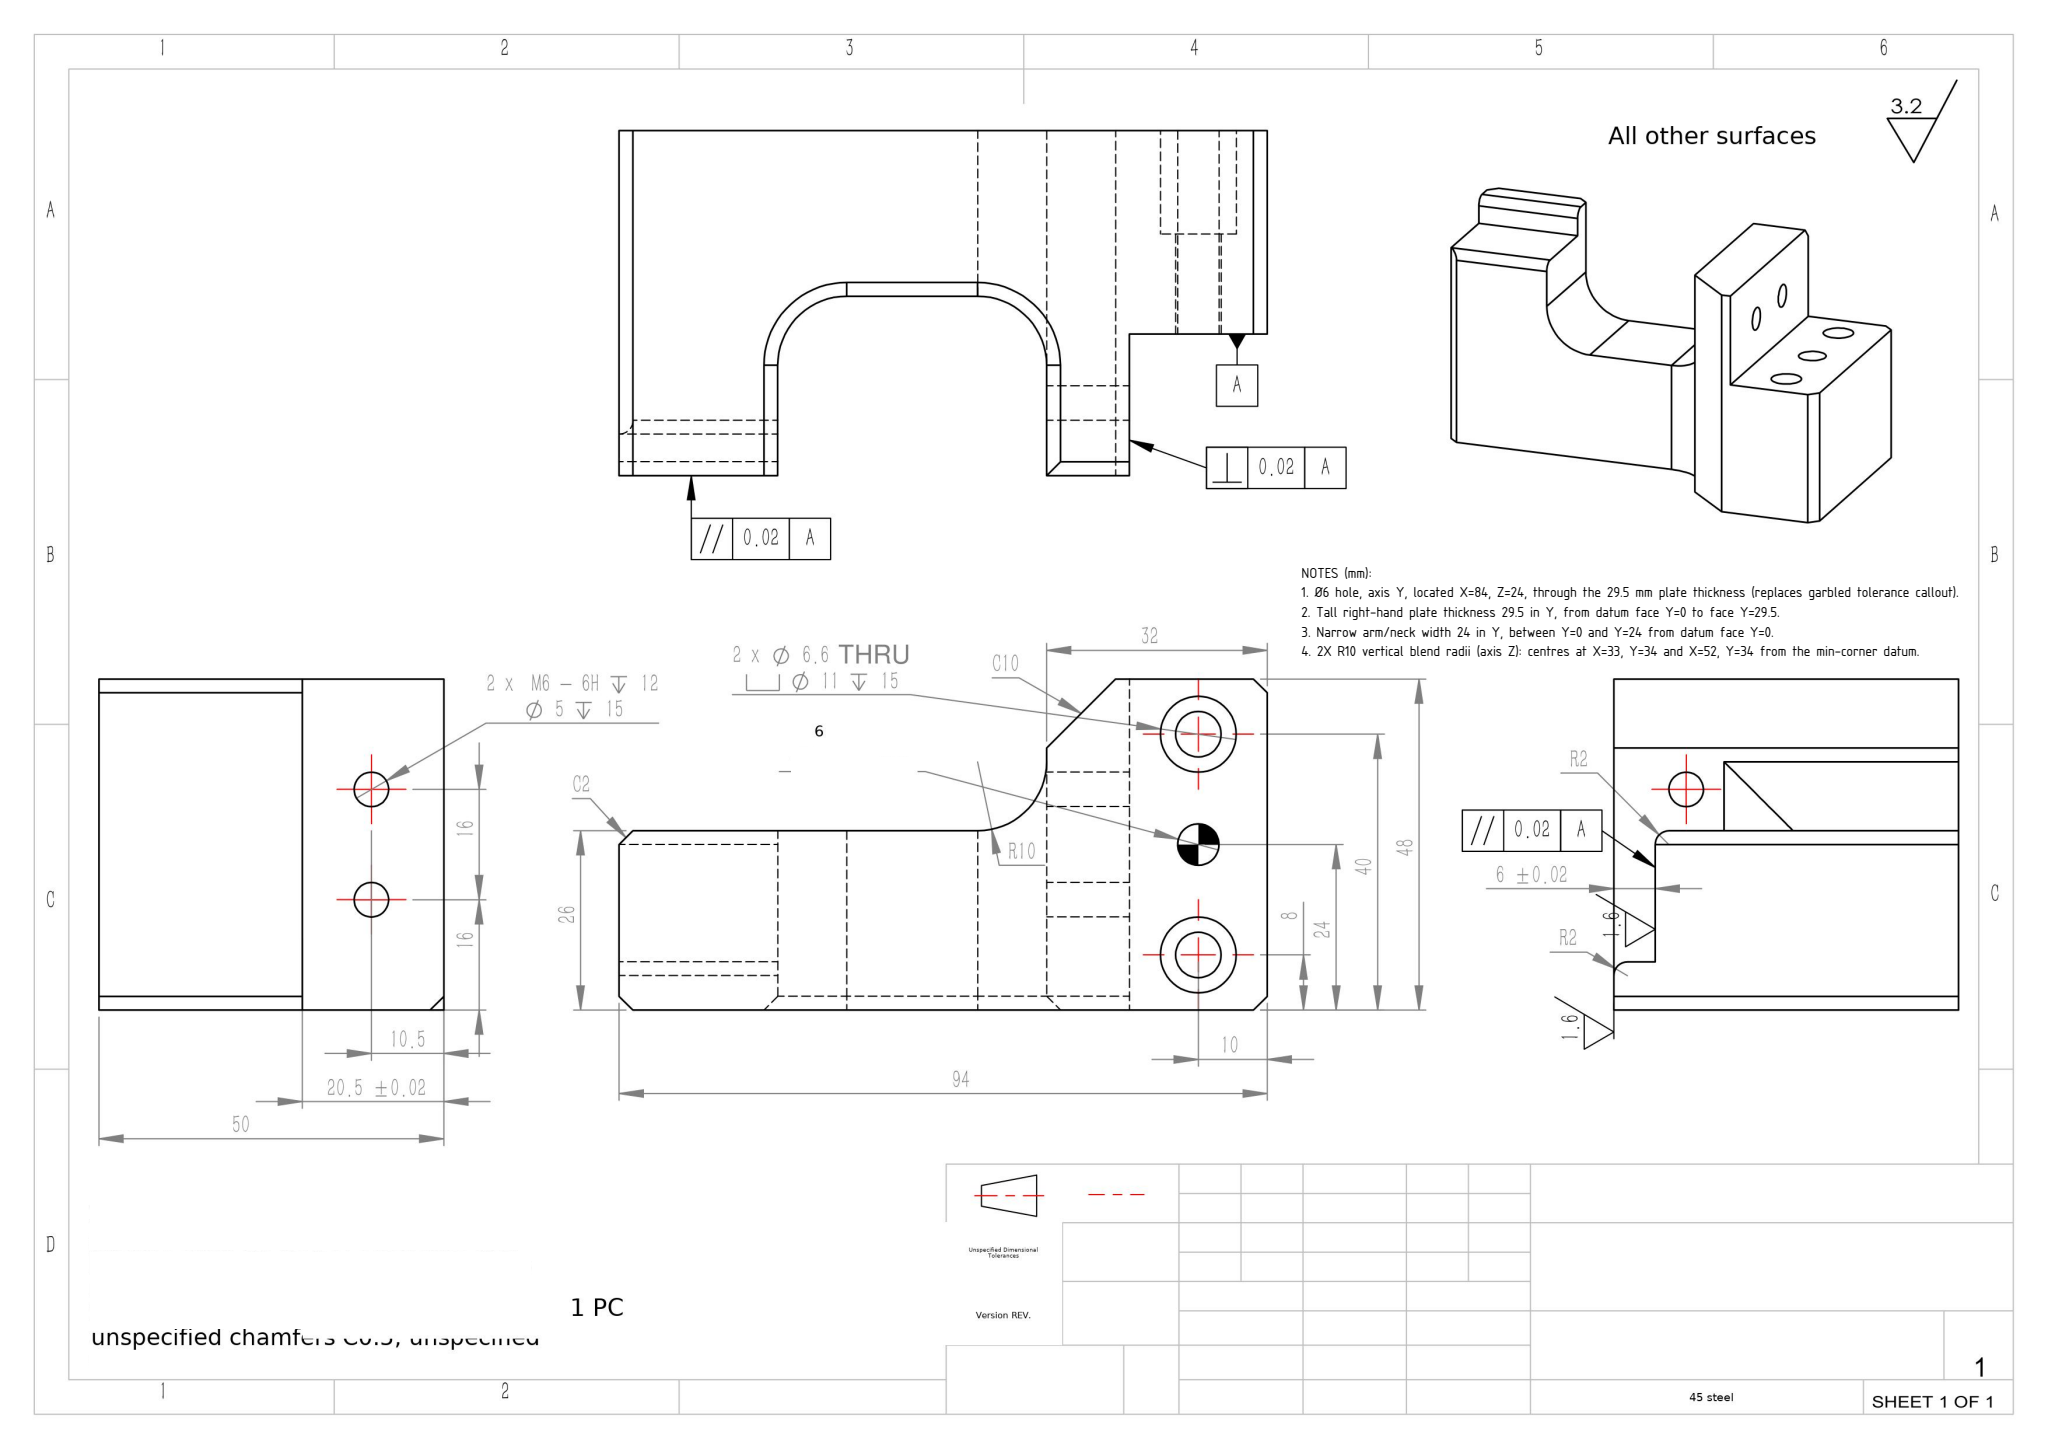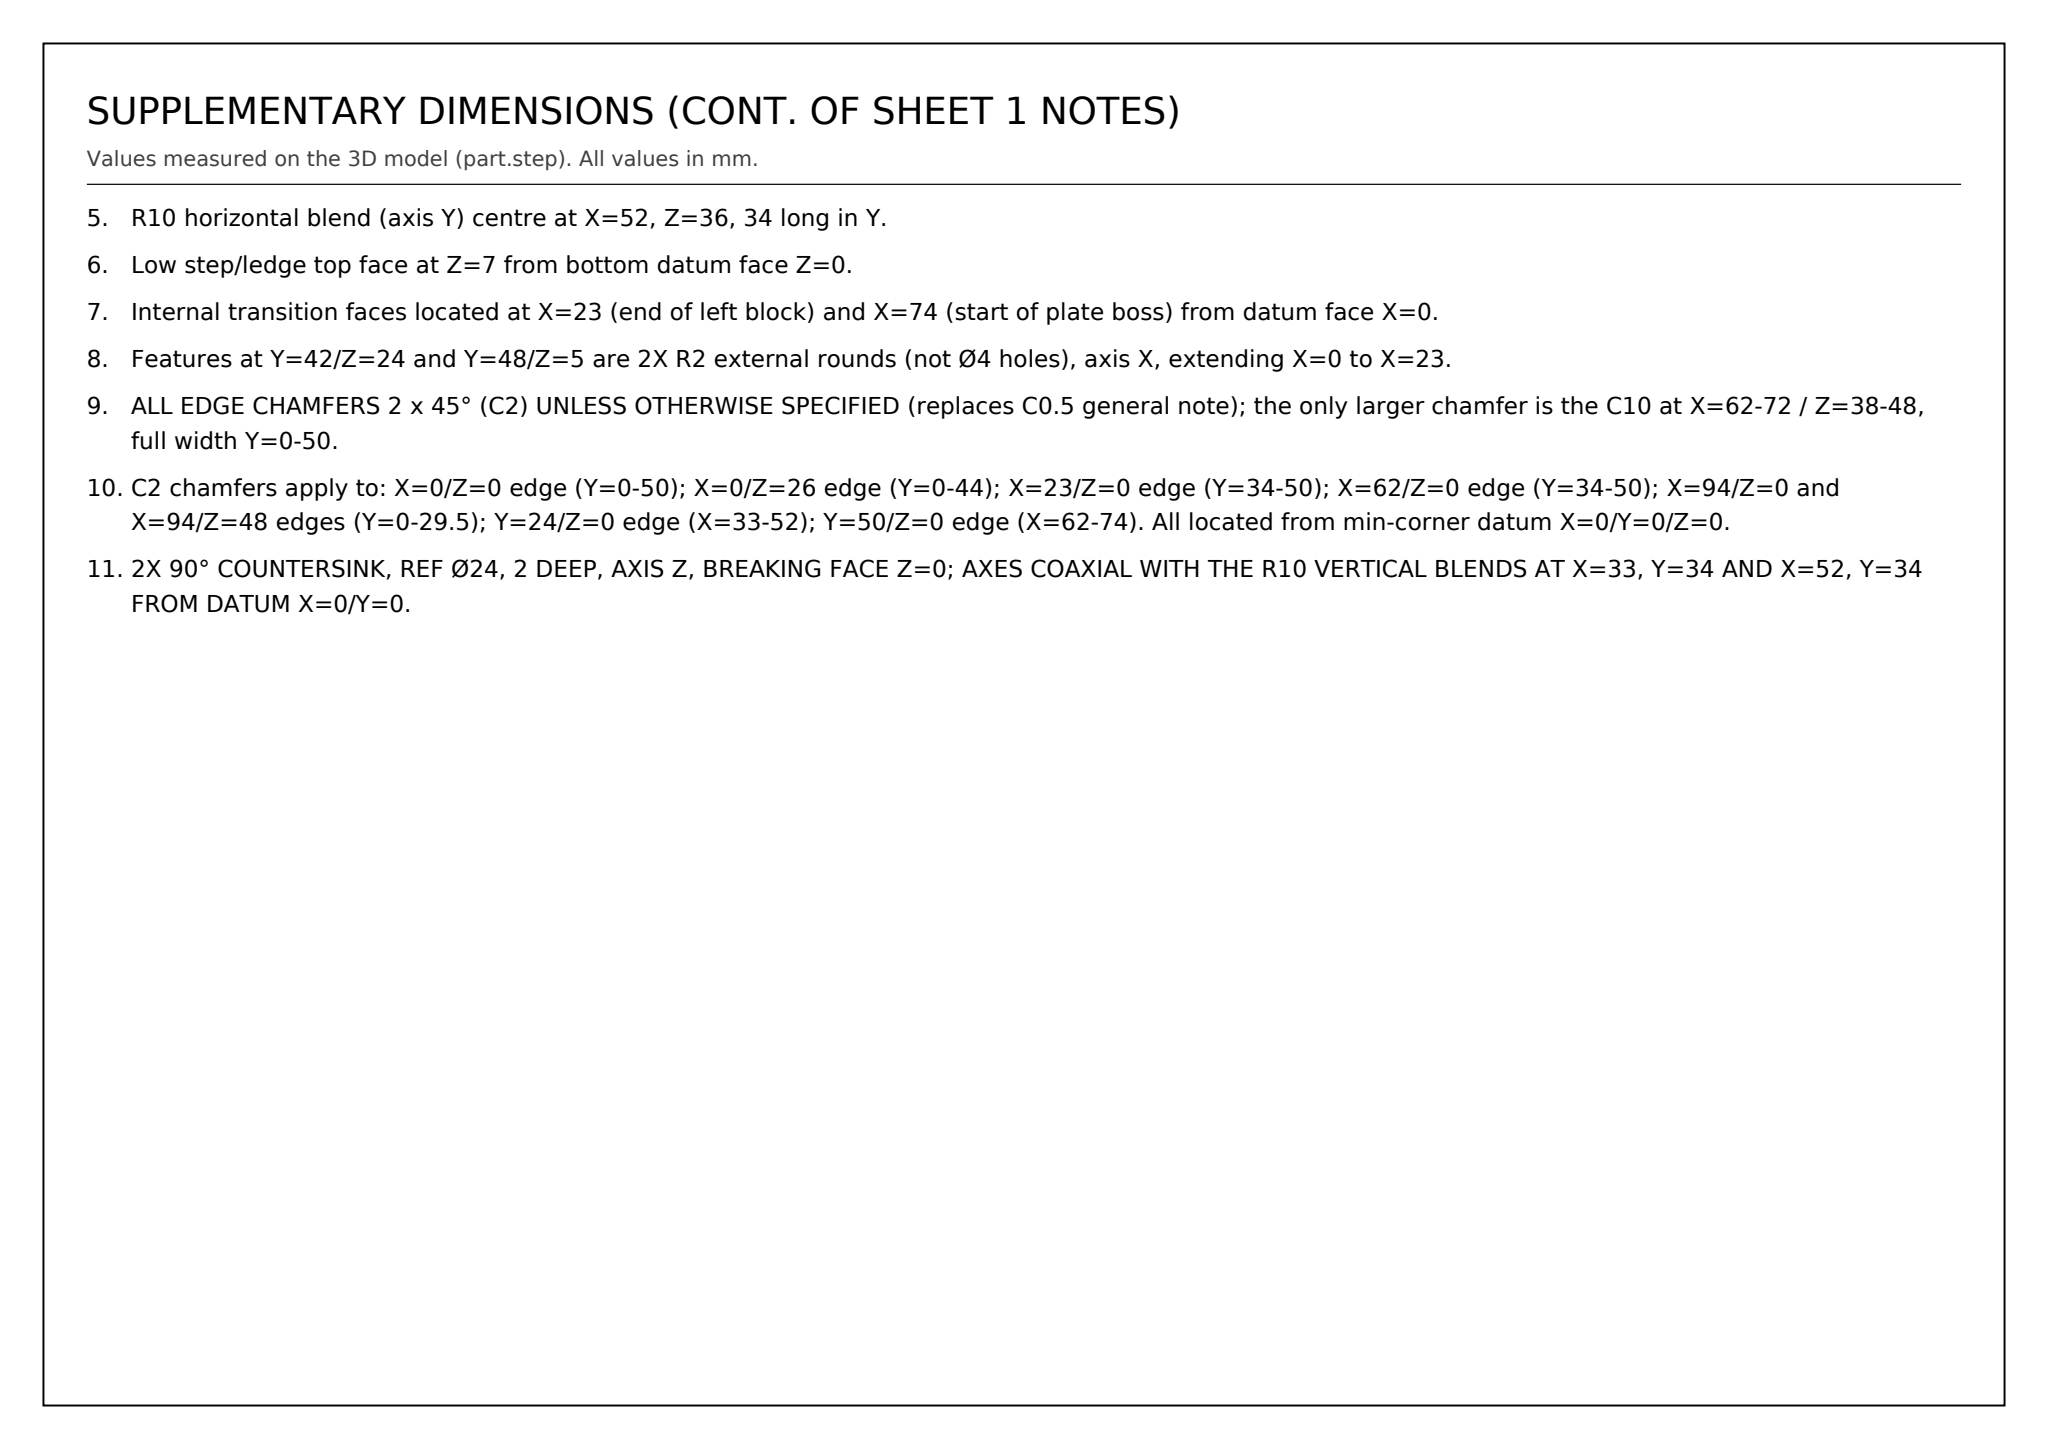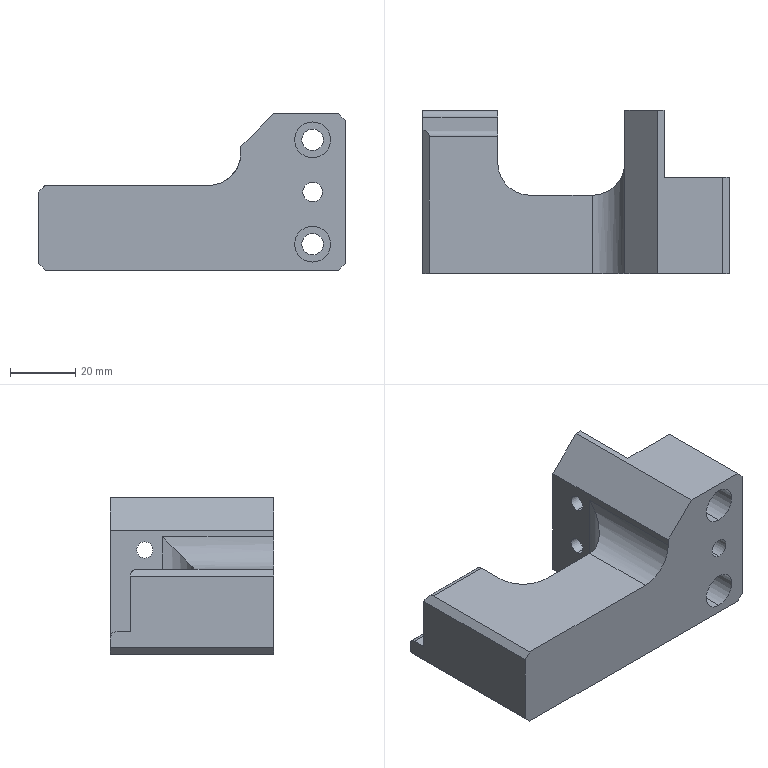Part | SolidWorks | mm | 1 solid | 47 faces | box 94 x 50 x 48 mm | volume 102278 mm3 | plane 26 | cylinder 19 | cone 2 | commonest cylinder face diameters 5 x4 11 x4 6.6 x4 20 x3 6 x2 4 x2
Drawing notes:
Ø6 hole, axis Y, located X=84, Z=24, through the 29.5 mm plate thickness (replaces garbled tolerance callout). | from the solid: cylinder dia 6.0 axis y at [84,null,24] length 29.5
Tall right-hand plate thickness 29.5 in Y, from datum face Y=0 to face Y=29.5. | from the solid: axis_planes y=0.0 and y=29.5; dia 6.0 y-cylinder length 29.5
Narrow arm/neck width 24 in Y, between Y=0 and Y=24 from datum face Y=0. | from the solid: Datum face y=0 spans x 0-94, z 0-48; the arm is bounded by plane y=24 (extent x 33-52, z 2-26), and the two vertical R10 concave blends (axis z, dia 20) at X=33,Y=34 and X=52,Y=34 are tangent to that y=24 face, so the neck runs Y=0 to Y=24 (width 24), not Y=24 to Y=44.
2X R10 vertical blend radii (axis Z): centres at X=33, Y=34 and X=52, Y=34 from the min-corner datum. | from the solid: cylinders dia 20.0 axis z at [33,34] L=24 and [52,34] L=34
R10 horizontal blend (axis Y) centre at X=52, Z=36, 34 long in Y. | from the solid: cylinder dia 20.0 axis y at [52,null,36] length 34
Low step/ledge top face at Z=7 from bottom datum face Z=0. | from the solid: axis_plane z=7.0
Internal transition faces located at X=23 (end of left block) and X=74 (start of plate boss) from datum face X=0. | from the solid: axis_planes x=23.0 and x=74.0 (also x=62.0)
Features at Y=42/Z=24 and Y=48/Z=5 are 2X R2 external rounds (not Ø4 holes), axis X, extending X=0 to X=23. | from the solid: cylinders: convex arc (round/outer radius) dia 4.0, axis x, at (y=42,z=24) and (y=48,z=5), from 0.0 to 23.0, 90 deg
ALL EDGE CHAMFERS 2 x 45° (C2) UNLESS OTHERWISE SPECIFIED (replaces C0.5 general note); the only larger chamfer is the C10 at X=62-72 / Z=38-48, full width Y=0-50. | from the solid: inclined_planes: eight 45° faces of 2 mm size plus one of 10 mm size at bbox_from [62,0,38]
C2 chamfers apply to: X=0/Z=0 edge (Y=0-50); X=0/Z=26 edge (Y=0-44); X=23/Z=0 edge (Y=34-50); X=62/Z=0 edge (Y=34-50); X=94/Z=0 and X=94/Z=48 edges (Y=0-29.5); Y=24/Z=0 edge (X=33-52); Y=50/Z=0 edge (X=62-74). All located from min-corner datum X=0/Y=0/Z=0. | from the solid: inclined_planes 45° entries bbox_from [0,0,0],[0,0,24],[21,34,0],[62,34,0],[92,0,0],[92,0,46],[33,22,0],[62,48,0], each 2 mm size
2X 90° COUNTERSINK, REF Ø24, 2 DEEP, AXIS Z, BREAKING FACE Z=0; AXES COAXIAL WITH THE R10 VERTICAL BLENDS AT X=33, Y=34 AND X=52, Y=34 FROM DATUM X=0/Y=0. | from the solid: cones[90.0, ref_dia 24] bbox_from [21,22,0] and [52,22,0], size [12,12,2]